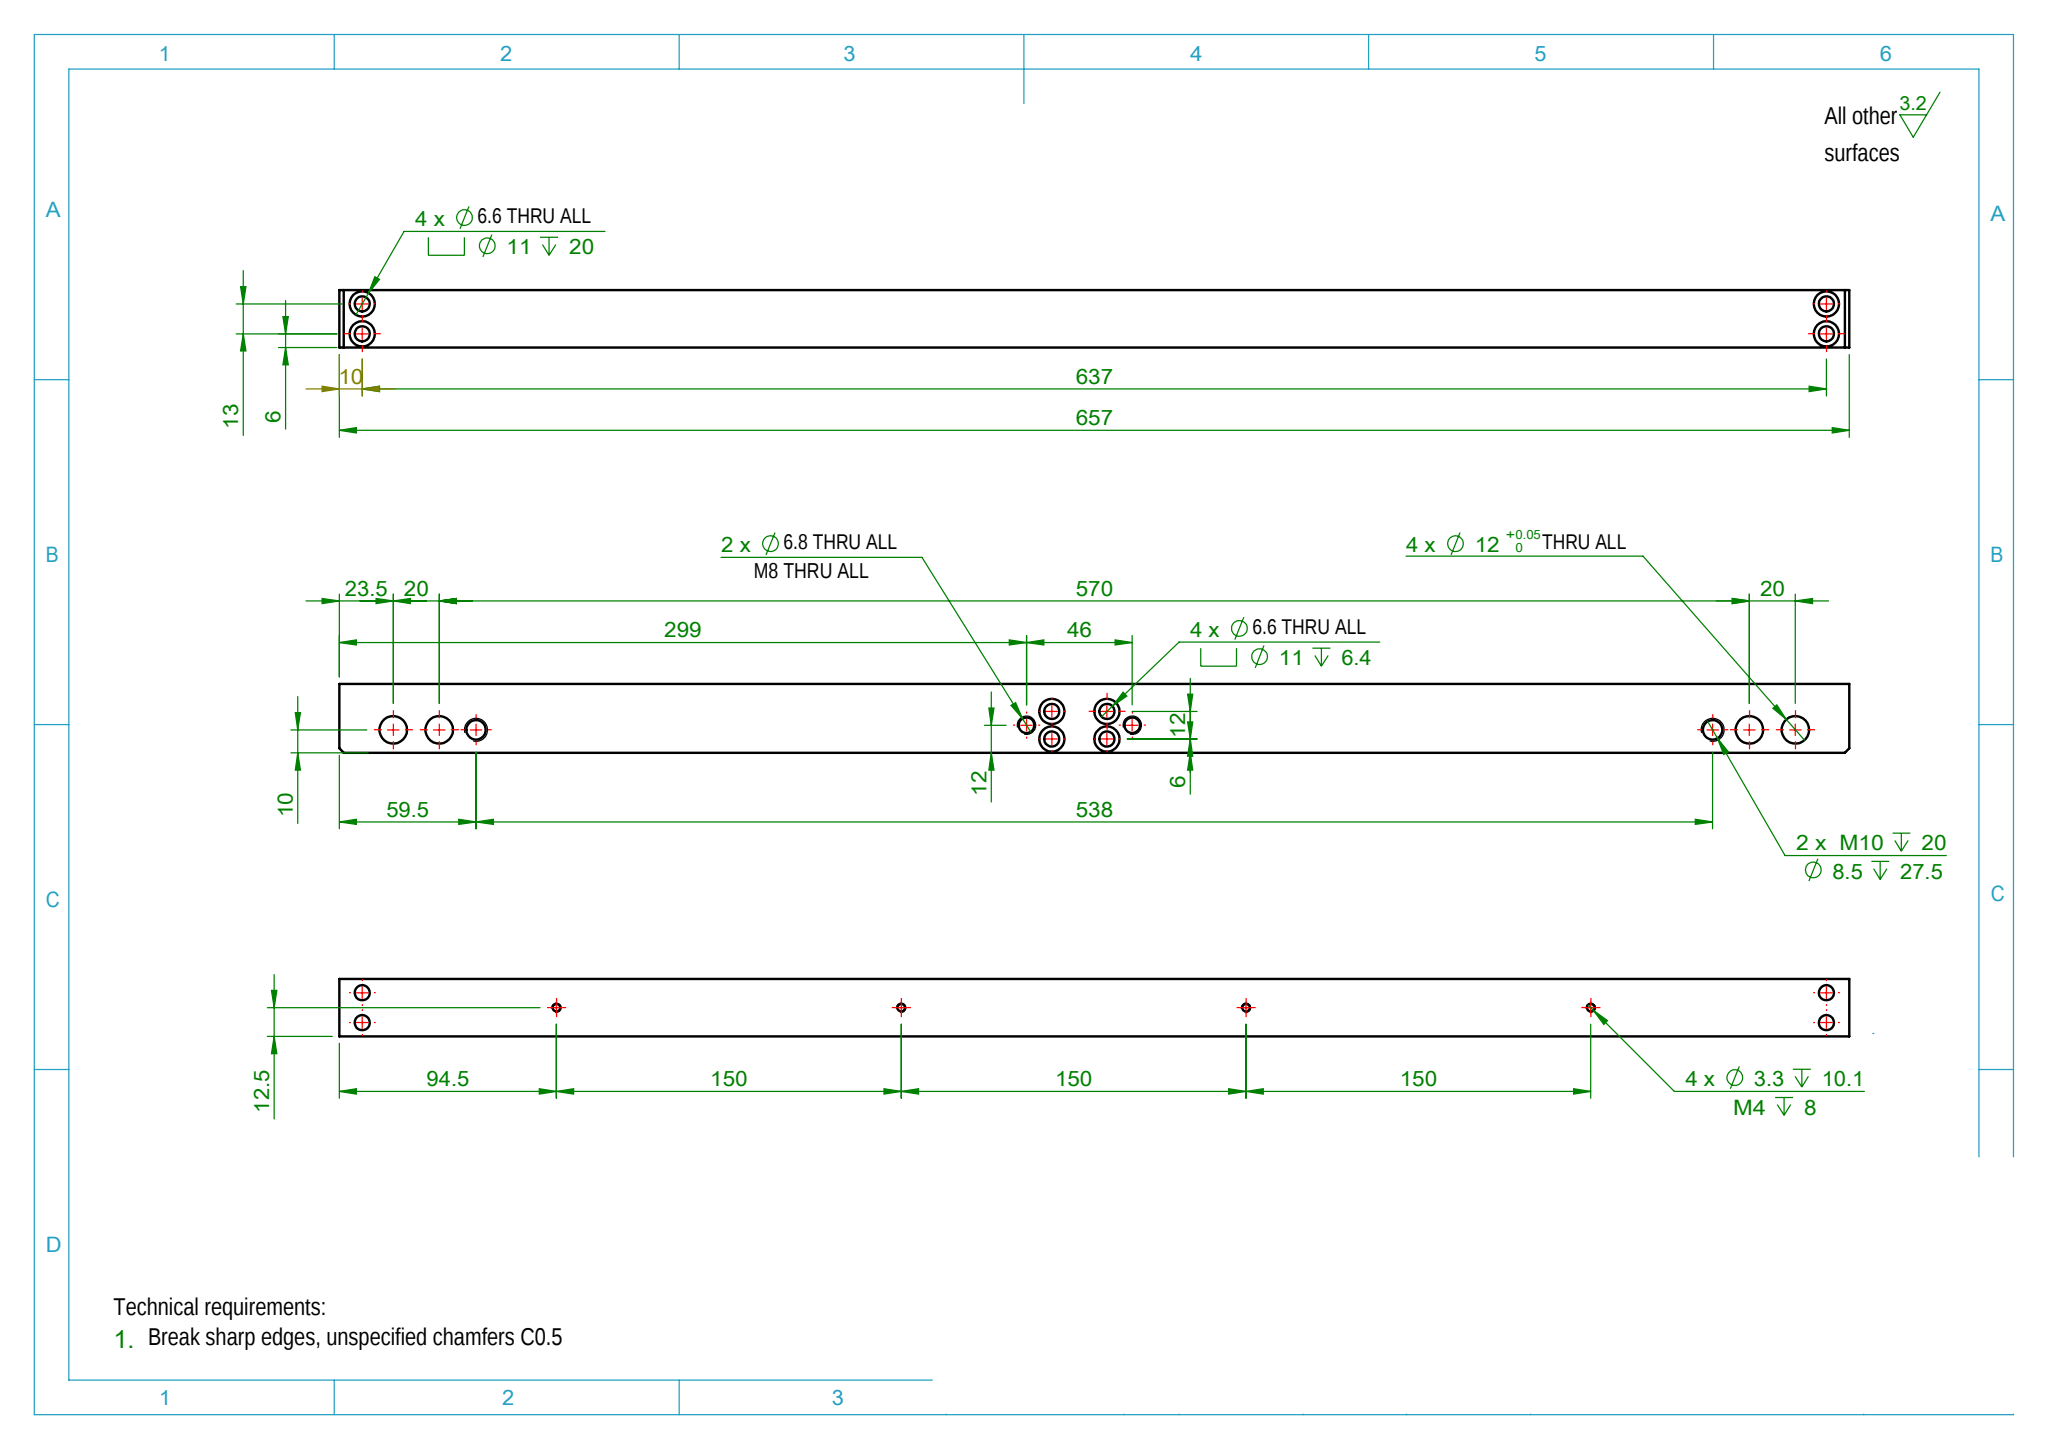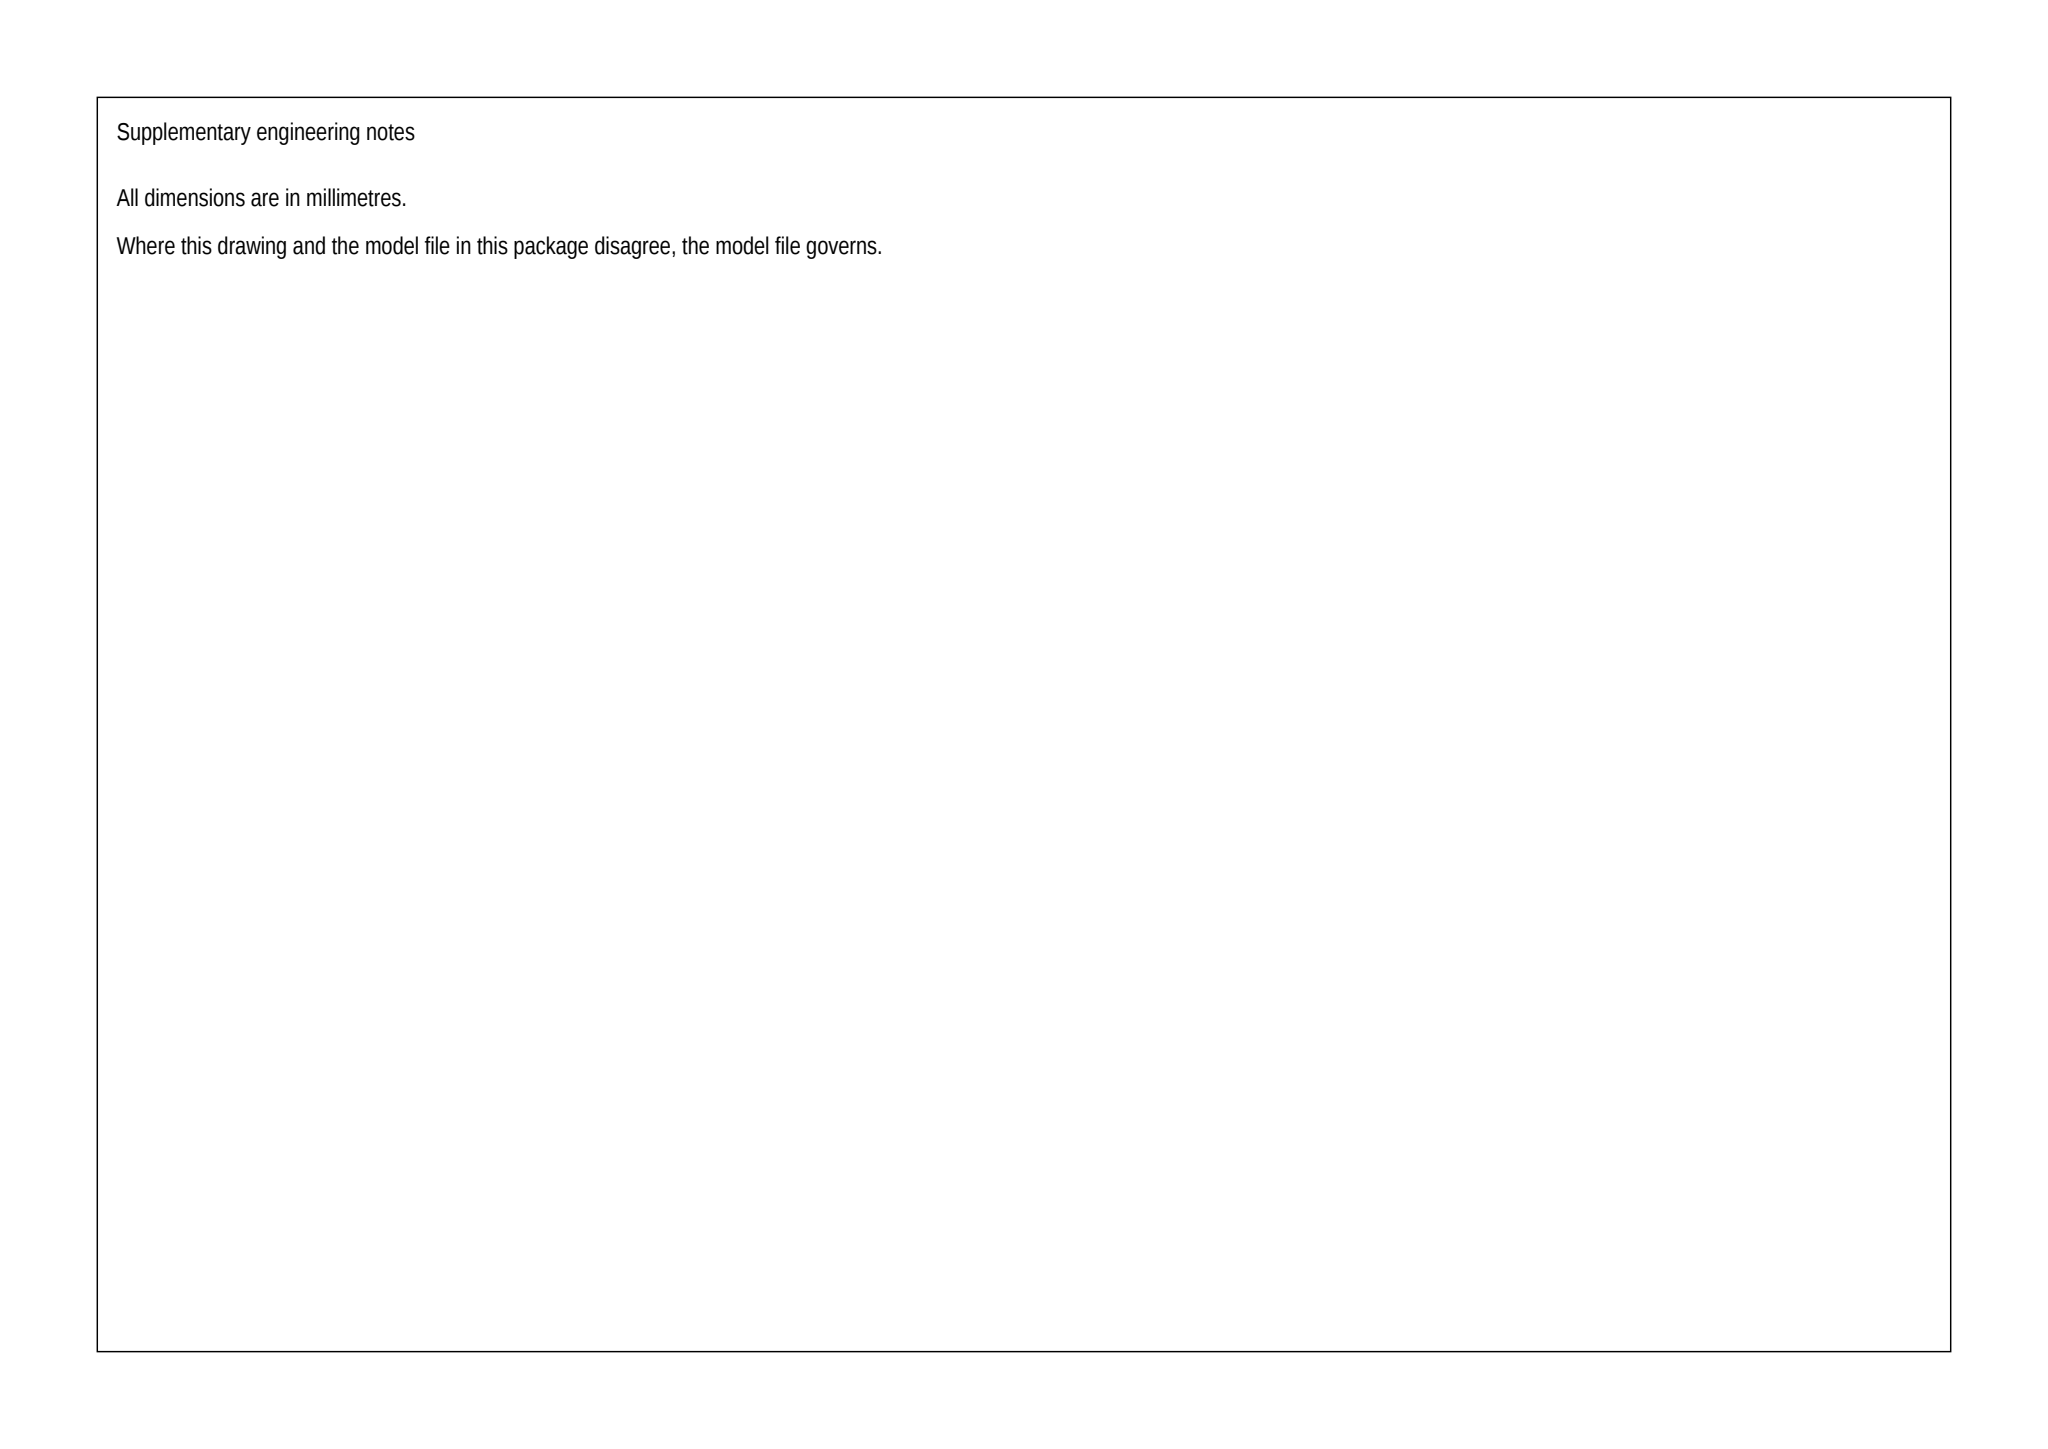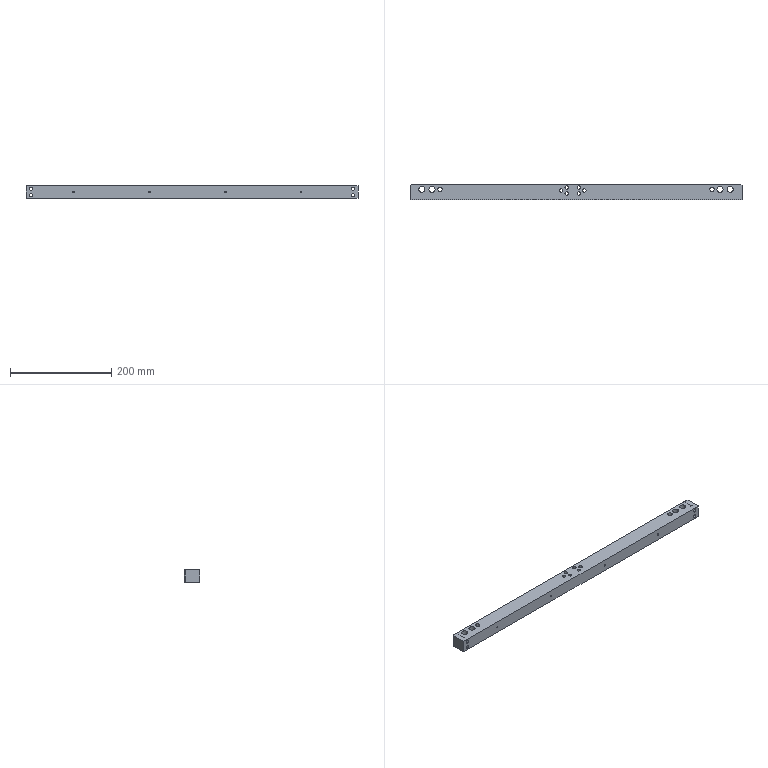Part | SolidWorks | mm | 1 solid | 80 faces | box 657 x 30 x 25 mm | volume 462381 mm3 | cylinder 56 | plane 16 | cone 8 | commonest cylinder face diameters 11 x16 6.6 x16 3.3 x8 12 x8 6.8 x4 8.5 x4
build123d program:
from build123d import *

# Parameters (mm, degrees)
SKETCH1_W                                       = 25
SKETCH1_H                                       = 30
BOSS_EXTRUDE1_DEPTH                             = 657
F_12_0_12_DIAMETER_HOLE1_D                      = 12
M10_TAPPED_HOLE1_D                              = 8.5
M10_TAPPED_HOLE1_DEPTH                          = 27.5
M10_TAPPED_HOLE1_TIP                            = 2.554
M6_HEX_SOCKET_HEAD_CAP_SCREW_CBORE1_D           = 6.6
M6_HEX_SOCKET_HEAD_CAP_SCREW_CBORE1_CBORE_D     = 11
M6_HEX_SOCKET_HEAD_CAP_SCREW_CBORE1_CBORE_DEPTH = 20
M4_TAPPED_HOLE1_D                               = 3.3
M4_TAPPED_HOLE1_DEPTH                           = 10.1
M4_TAPPED_HOLE1_TIP                             = 0.9914
M6_HEX_SOCKET_HEAD_CAP_SCREW_CBORE2_D           = 6.6
M6_HEX_SOCKET_HEAD_CAP_SCREW_CBORE2_CBORE_D     = 11
M6_HEX_SOCKET_HEAD_CAP_SCREW_CBORE2_CBORE_DEPTH = 6.4
M8_TAPPED_HOLE1_D                               = 6.8
CHAMFER2_SIZE                                   = 2


with BuildPart() as part:
    # Sketch1 → Boss-Extrude1 (new body)
    with BuildSketch(Plane(origin=(0, 0, 0), x_dir=(0, 0, -1), z_dir=(1, 0, 0))):
        with Locations((12.5, 15)):
            Rectangle(SKETCH1_W, SKETCH1_H)
    extrude(amount=BOSS_EXTRUDE1_DEPTH)

    # 12.0 _12_ Diameter Hole1 (through all)
    with Locations(Plane.XY):
        with Locations((23.5, 20), (43.5, 20), (613.5, 20), (633.5, 20)):
            Hole(F_12_0_12_DIAMETER_HOLE1_D / 2)

    # M10 Tapped Hole1
    with Locations(Plane(origin=(0, 0, -25), x_dir=(-1, 0, 0), z_dir=(0, 0, -1))):
        with Locations((-597.5, 20), (-59.5, 20)):
            Hole(M10_TAPPED_HOLE1_D / 2, depth=M10_TAPPED_HOLE1_DEPTH)
            with Locations((0, 0, -(M10_TAPPED_HOLE1_DEPTH + M10_TAPPED_HOLE1_TIP / 2))):  # 118° drill point
                Cone(0, M10_TAPPED_HOLE1_D / 2, M10_TAPPED_HOLE1_TIP, mode=Mode.SUBTRACT)

    # M6 Hex Socket Head Cap Screw CBORE1 (through all)
    with Locations(Plane(origin=(0, 30, 0), x_dir=(1, 0, 0), z_dir=(0, 1, 0))):
        with Locations((10, 19), (10, 6), (647, 19), (647, 6)):
            CounterBoreHole(M6_HEX_SOCKET_HEAD_CAP_SCREW_CBORE1_D / 2, M6_HEX_SOCKET_HEAD_CAP_SCREW_CBORE1_CBORE_D / 2, M6_HEX_SOCKET_HEAD_CAP_SCREW_CBORE1_CBORE_DEPTH)

    # M4 Tapped Hole1
    with Locations(Plane(origin=(0, 0, 0), x_dir=(-1, 0, 0), z_dir=(0, -1, 0))):
        with Locations((-544.5, 12.5), (-394.5, 12.5), (-244.5, 12.5), (-94.5, 12.5)):
            Hole(M4_TAPPED_HOLE1_D / 2, depth=M4_TAPPED_HOLE1_DEPTH)
            with Locations((0, 0, -(M4_TAPPED_HOLE1_DEPTH + M4_TAPPED_HOLE1_TIP / 2))):  # 118° drill point
                Cone(0, M4_TAPPED_HOLE1_D / 2, M4_TAPPED_HOLE1_TIP, mode=Mode.SUBTRACT)

    # M6 Hex Socket Head Cap Screw CBORE2 (through all)
    with Locations(Plane(origin=(0, 0, -25), x_dir=(-1, 0, 0), z_dir=(0, 0, -1))):
        with Locations((-334, 24), (-310, 24), (-334, 12), (-310, 12)):
            CounterBoreHole(M6_HEX_SOCKET_HEAD_CAP_SCREW_CBORE2_D / 2, M6_HEX_SOCKET_HEAD_CAP_SCREW_CBORE2_CBORE_D / 2, M6_HEX_SOCKET_HEAD_CAP_SCREW_CBORE2_CBORE_DEPTH)

    # M8 Tapped Hole1 (through all)
    with Locations(Plane(origin=(0, 0, -25), x_dir=(-1, 0, 0), z_dir=(0, 0, -1))):
        with Locations((-345, 18), (-299, 18)):
            Hole(M8_TAPPED_HOLE1_D / 2)

    # Chamfer2
    chamfer2_edges = [part.edges().sort_by_distance(p)[0] for p in [
        (657, 30, -12.5),
        (0, 30, -12.5),
    ]]
    chamfer(chamfer2_edges, length=CHAMFER2_SIZE)


solid = part.part